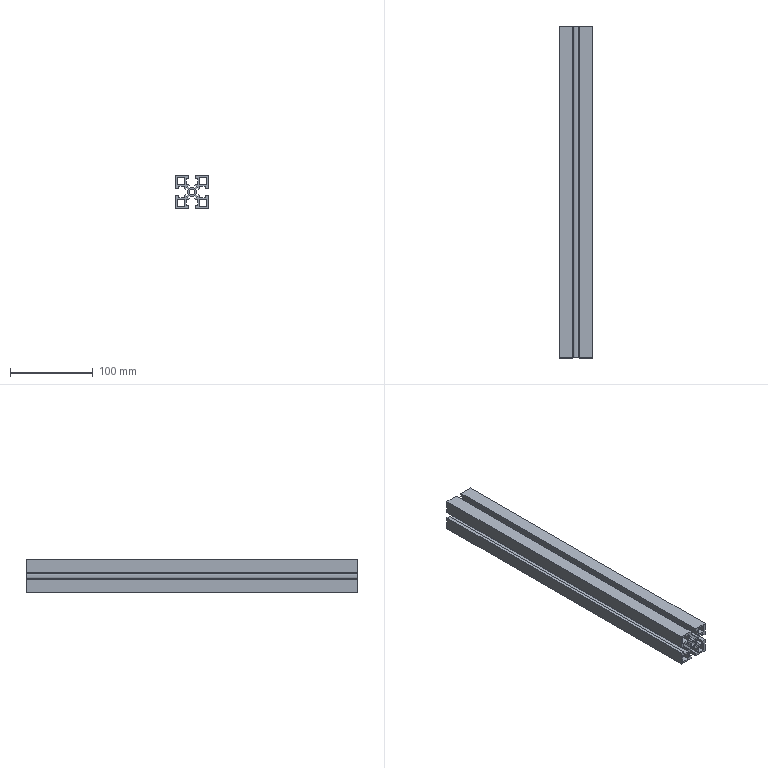Component | SolidWorks | AluminumProfile360-1 | 1 solid | 89 faces | box 40 x 400 x 40 mm | volume 232030 mm3 | plane 82 | cylinder 7 | commonest cylinder face diameters 10.5 x5 6.8 x2 | material 6061 Alloy
build123d program:
from build123d import *

# Parameters (mm, degrees)
SKETCH1_W                  = 40
SKETCH1_H                  = 40
EXTRUDE1_DEPTH             = 1640
CUT_EXTRUDE1_DEPTH         = 1641.975
SKETCH3_R                  = 3.4
CUT_EXTRUDE2_DEPTH         = 1641.975
CIRPATTERN1_COUNT          = 4
EXTRUDE2_DEPTH             = 1641.975
CIRPATTERN2_COUNT          = 4
SKETCH5_W                  = 9
SKETCH5_H                  = 9
EXTRUDE3_DEPTH             = 1641.975
CIRPATTERN3_COUNT          = 4
M8X1_25_TAPPED_HOLE3_D     = 6.8
M8X1_25_TAPPED_HOLE3_DEPTH = 19.75
M8X1_25_TAPPED_HOLE3_TIP   = 2.043
SKETCH9_W                  = 177.591
SKETCH9_H                  = 2021.808
CUT_EXTRUDE3_DEPTH         = 1641.975


with BuildPart() as part:
    # Sketch1 → Extrude1 (new body)
    with BuildSketch(Plane.XY):
        with Locations((20, 20)):
            Rectangle(SKETCH1_W, SKETCH1_H)
    extrude(amount=EXTRUDE1_DEPTH)

    # Sketch2 → Cut-Extrude1 (cut, through all)
    with BuildSketch(Plane.XY.offset(1640)):
        Polygon((16, 40), (16, 36), (13, 36), (13, 29), (27, 29), (27, 36), (24, 36), (24, 40), align=None)
    cut_extrude1 = extrude(amount=-CUT_EXTRUDE1_DEPTH, mode=Mode.SUBTRACT)

    # Sketch3 → Cut-Extrude2 (cut, through all)
    with BuildSketch(Plane.XY.offset(1640)):
        with Locations((20, 20)):
            Circle(SKETCH3_R)
    extrude(amount=-CUT_EXTRUDE2_DEPTH, mode=Mode.SUBTRACT)

    # CirPattern1: Cut-Extrude1 ×4 about axis
    cirpattern1_axis = Axis((20, 20, 0), (0, 0, 1))
    for i in range(1, CIRPATTERN1_COUNT):
        add(cut_extrude1.rotate(cirpattern1_axis, i * 360 / CIRPATTERN1_COUNT), mode=Mode.SUBTRACT)

    # Sketch4 → Extrude2 (cut, through all)
    with BuildSketch(Plane.XY.offset(1640)):
        with BuildLine():
            Line((15.75, 29), (16.457, 28.293))
            Line((16.457, 28.293), (14.806, 26.641))
            Line((14.806, 26.641), (17.082, 24.365))
            ThreePointArc((17.082, 24.365), (20, 25.25), (22.918, 24.365))
            Line((22.918, 24.365), (25.194, 26.641))
            Line((25.194, 26.641), (23.543, 28.293))
            Line((23.543, 28.293), (24.25, 29))
            Line((24.25, 29), (15.75, 29))
        make_face()
    extrude2 = extrude(amount=-EXTRUDE2_DEPTH, mode=Mode.SUBTRACT)

    # CirPattern2: Extrude2 ×4 about axis
    cirpattern2_axis = Axis((20, 20, 0), (0, 0, 1))
    for i in range(1, CIRPATTERN2_COUNT):
        add(extrude2.rotate(cirpattern2_axis, i * 360 / CIRPATTERN2_COUNT), mode=Mode.SUBTRACT)

    # Sketch5 → Extrude3 (cut, through all)
    with BuildSketch(Plane.XY.offset(1640)):
        with Locations((6.5, 33.5)):
            Rectangle(SKETCH5_W, SKETCH5_H)
    extrude3 = extrude(amount=-EXTRUDE3_DEPTH, mode=Mode.SUBTRACT)

    # CirPattern3: Extrude3 ×4 about axis
    cirpattern3_axis = Axis((20, 20, 0), (0, 0, 1))
    for i in range(1, CIRPATTERN3_COUNT):
        add(extrude3.rotate(cirpattern3_axis, i * 360 / CIRPATTERN3_COUNT), mode=Mode.SUBTRACT)

    # M8x1.25 Tapped Hole3
    with Locations(Plane(origin=(20, 20, 1640), x_dir=(1, 0, 0), z_dir=(0, 0, 1))):
        with Locations((0, 0)):
            Hole(M8X1_25_TAPPED_HOLE3_D / 2, depth=M8X1_25_TAPPED_HOLE3_DEPTH)
            with Locations((0, 0, -(M8X1_25_TAPPED_HOLE3_DEPTH + M8X1_25_TAPPED_HOLE3_TIP / 2))):  # 118° drill point
                Cone(0, M8X1_25_TAPPED_HOLE3_D / 2, M8X1_25_TAPPED_HOLE3_TIP, mode=Mode.SUBTRACT)

    # Sketch9 → Cut-Extrude3 (cut, through all)
    with BuildSketch(Plane.XZ):
        with Locations((13.869, 1410.904)):
            Rectangle(SKETCH9_W, SKETCH9_H)
    extrude(amount=-CUT_EXTRUDE3_DEPTH, mode=Mode.SUBTRACT)


solid = part.part

# Placed as in the assembly
solid = solid.moved(Location((-968.352, -608.217, 359.715), (90, 0, 0)))